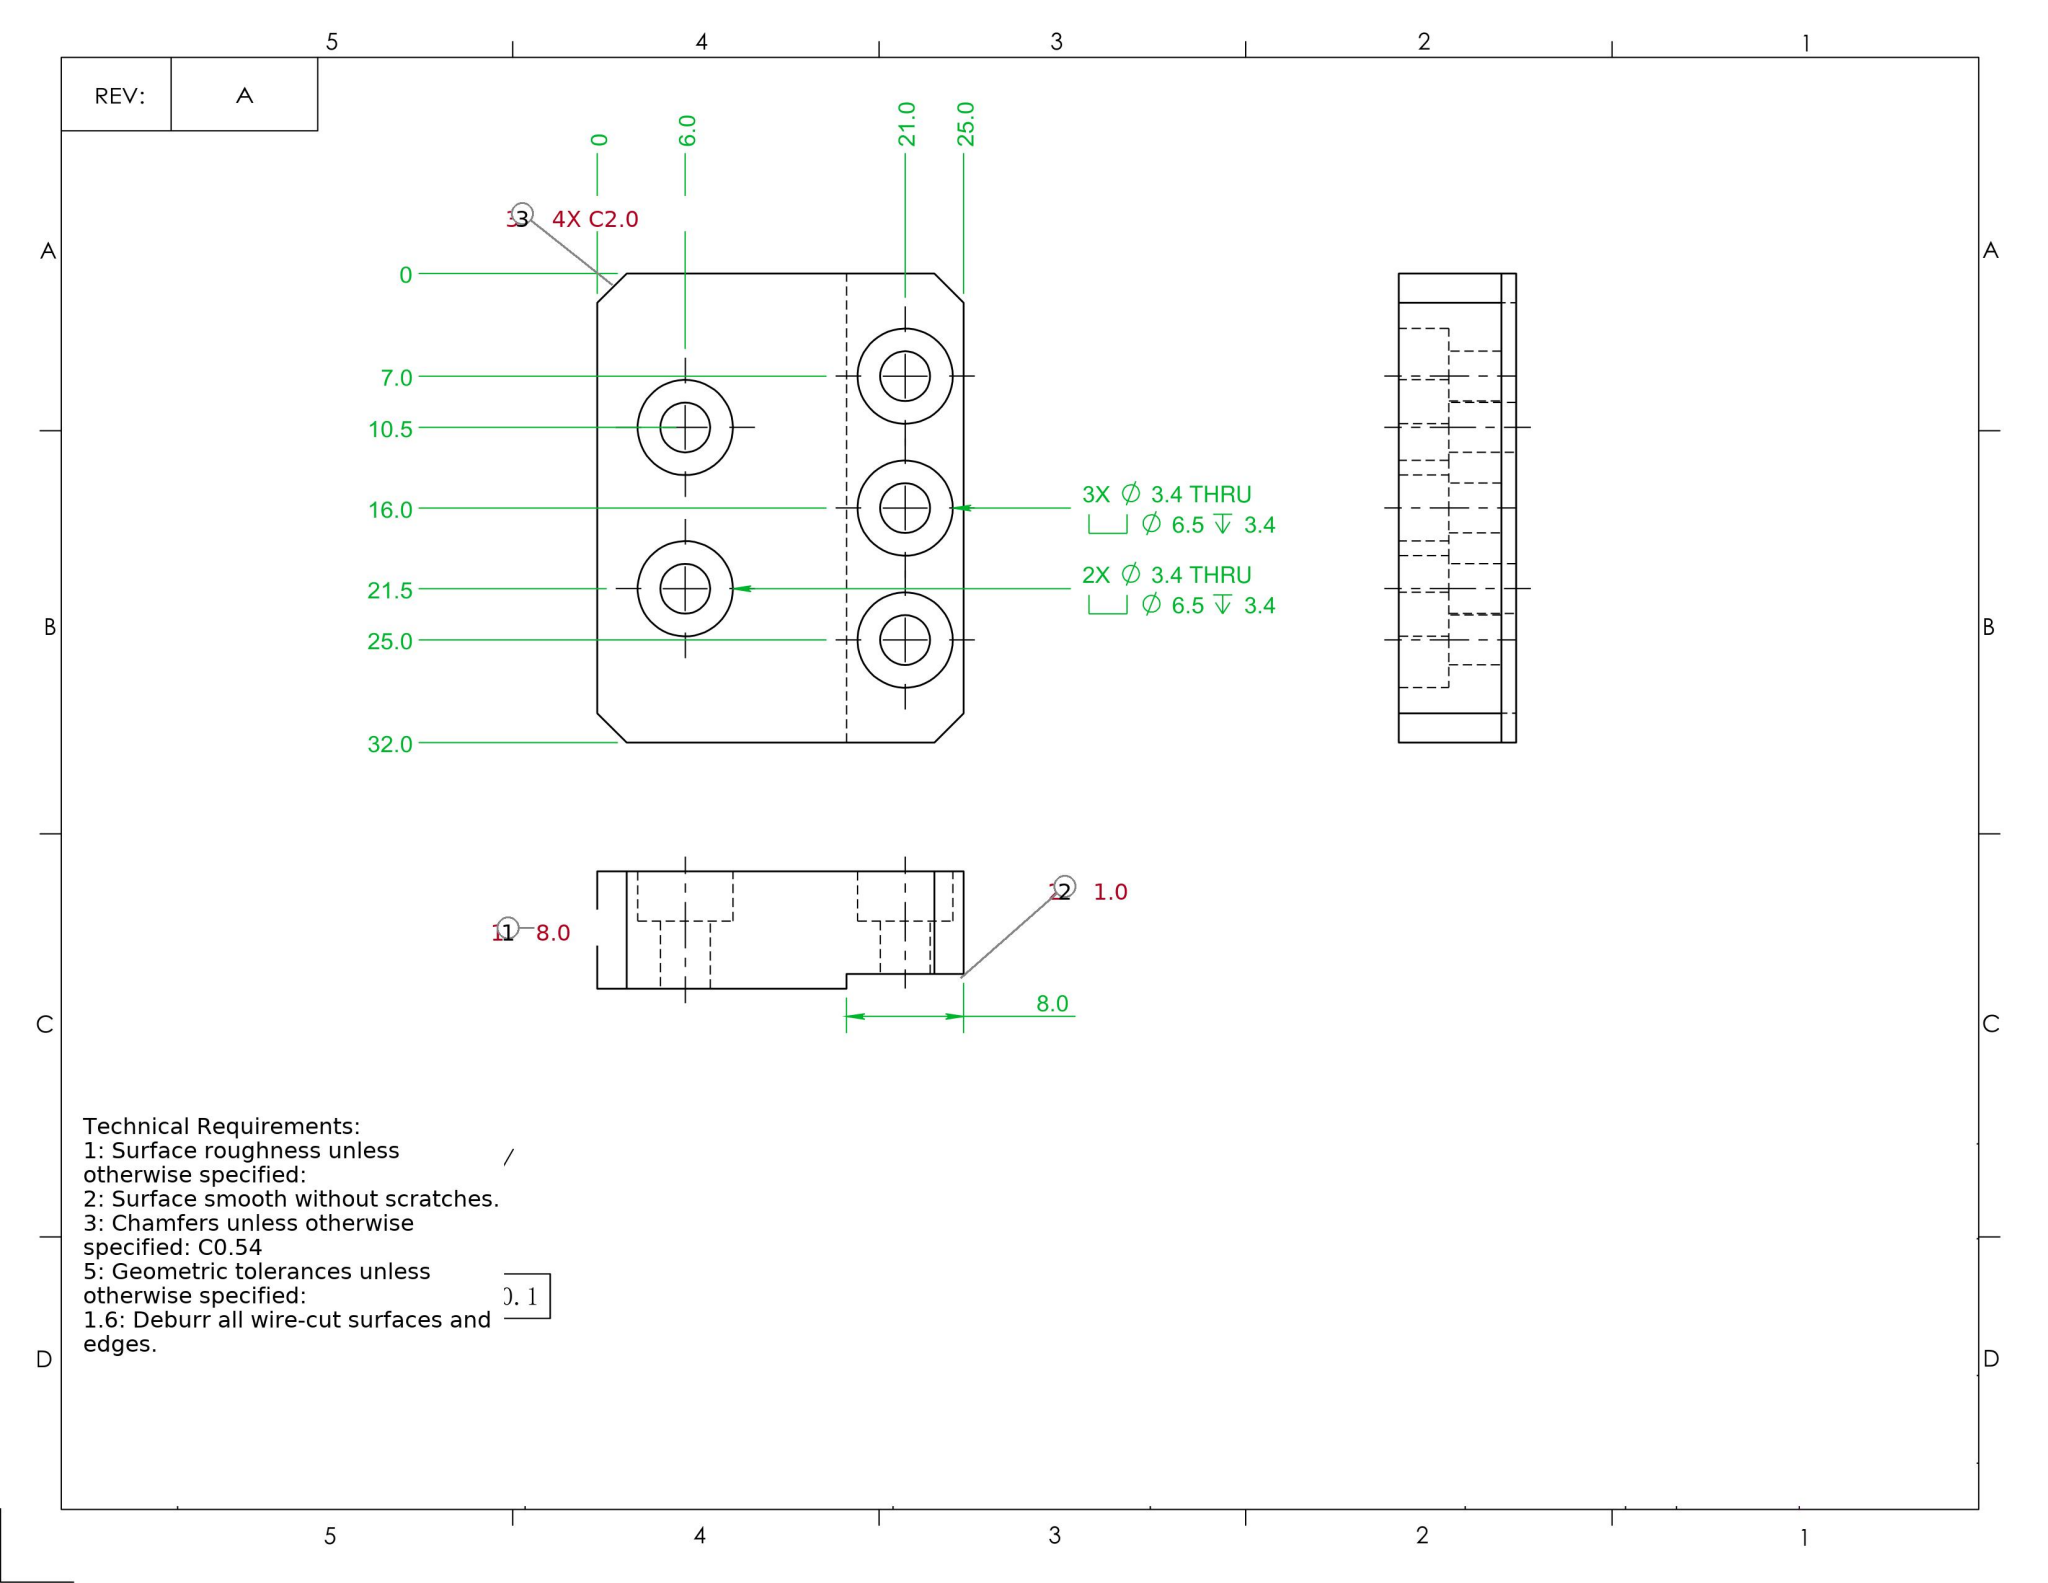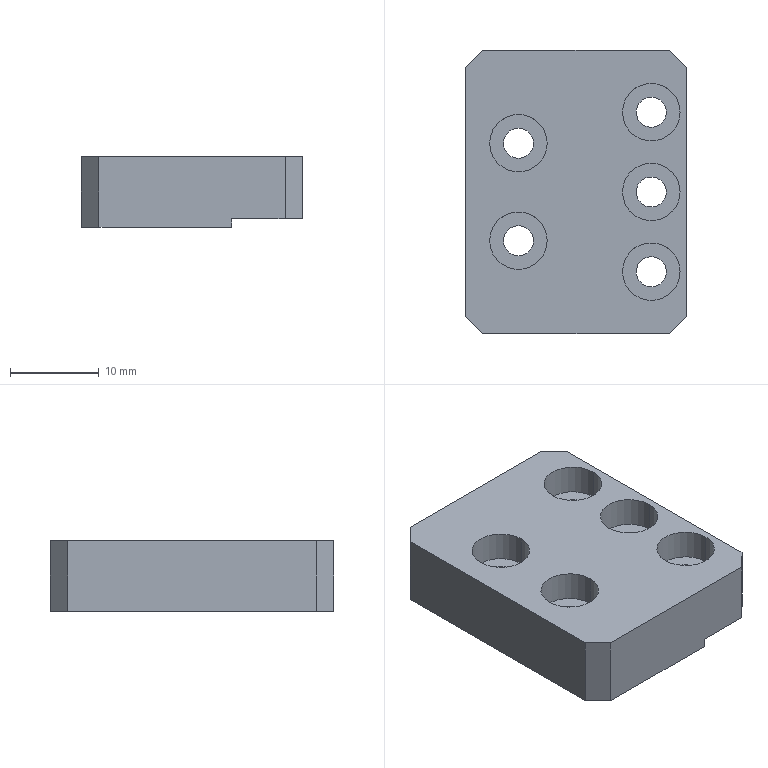Part | SolidWorks | mm | 1 solid | 37 faces | box 25 x 32 x 8 mm | volume 5338 mm3 | cylinder 20 | plane 17 | commonest cylinder face diameters 6.5 x10 3.4 x10
build123d program:
from build123d import *

# Parameters (mm, degrees)
SKETCH1_W                                       = 25
SKETCH1_H                                       = 32
BOSS_EXTRUDE1_DEPTH                             = 8
SKETCH4_W                                       = 8
SKETCH4_H                                       = 1
CUT_EXTRUDE3_DEPTH                              = 42.388
M3_HEX_SOCKET_HEAD_CAP_SCREW_CBORE1_D           = 3.4
M3_HEX_SOCKET_HEAD_CAP_SCREW_CBORE1_CBORE_D     = 6.5
M3_HEX_SOCKET_HEAD_CAP_SCREW_CBORE1_CBORE_DEPTH = 3.4
CHAMFER1_SIZE                                   = 2
CHAMFER2_SIZE                                   = 2
M3_HEX_SOCKET_HEAD_CAP_SCREW_CBORE2_D           = 3.4
M3_HEX_SOCKET_HEAD_CAP_SCREW_CBORE2_CBORE_D     = 6.5
M3_HEX_SOCKET_HEAD_CAP_SCREW_CBORE2_CBORE_DEPTH = 3.4


with BuildPart() as part:
    # Sketch1 → Boss-Extrude1 (new body)
    with BuildSketch(Plane.XY):
        with Locations((12.5, 16)):
            Rectangle(SKETCH1_W, SKETCH1_H)
    extrude(amount=BOSS_EXTRUDE1_DEPTH)

    # Sketch4 → Cut-Extrude3 (cut, through all)
    with BuildSketch(Plane(origin=(0, 32, 0), x_dir=(1, 0, 0), z_dir=(0, 1, 0))):
        with Locations((21, -0.5)):
            Rectangle(SKETCH4_W, SKETCH4_H)
    extrude(amount=-CUT_EXTRUDE3_DEPTH, mode=Mode.SUBTRACT)

    # M3 Hex Socket Head Cap Screw CBORE1 (through all)
    with Locations(Plane.XY.offset(8)):
        with Locations((21, 25), (21, 16), (21, 7)):
            CounterBoreHole(M3_HEX_SOCKET_HEAD_CAP_SCREW_CBORE1_D / 2, M3_HEX_SOCKET_HEAD_CAP_SCREW_CBORE1_CBORE_D / 2, M3_HEX_SOCKET_HEAD_CAP_SCREW_CBORE1_CBORE_DEPTH)

    # Chamfer1
    chamfer1_edges = [part.edges().sort_by_distance(p)[0] for p in [
        (25, 32, 4.5),
        (25, 0, 4.5),
    ]]
    chamfer(chamfer1_edges, length=CHAMFER1_SIZE)

    # Chamfer2
    chamfer2_edges = [part.edges().sort_by_distance(p)[0] for p in [
        (0, 32, 4),
        (0, 0, 4),
    ]]
    chamfer(chamfer2_edges, length=CHAMFER2_SIZE)

    # M3 Hex Socket Head Cap Screw CBORE2 (through all)
    with Locations(Plane.XY.offset(8)):
        with Locations((6, 21.5), (6, 10.5)):
            CounterBoreHole(M3_HEX_SOCKET_HEAD_CAP_SCREW_CBORE2_D / 2, M3_HEX_SOCKET_HEAD_CAP_SCREW_CBORE2_CBORE_D / 2, M3_HEX_SOCKET_HEAD_CAP_SCREW_CBORE2_CBORE_DEPTH)


solid = part.part